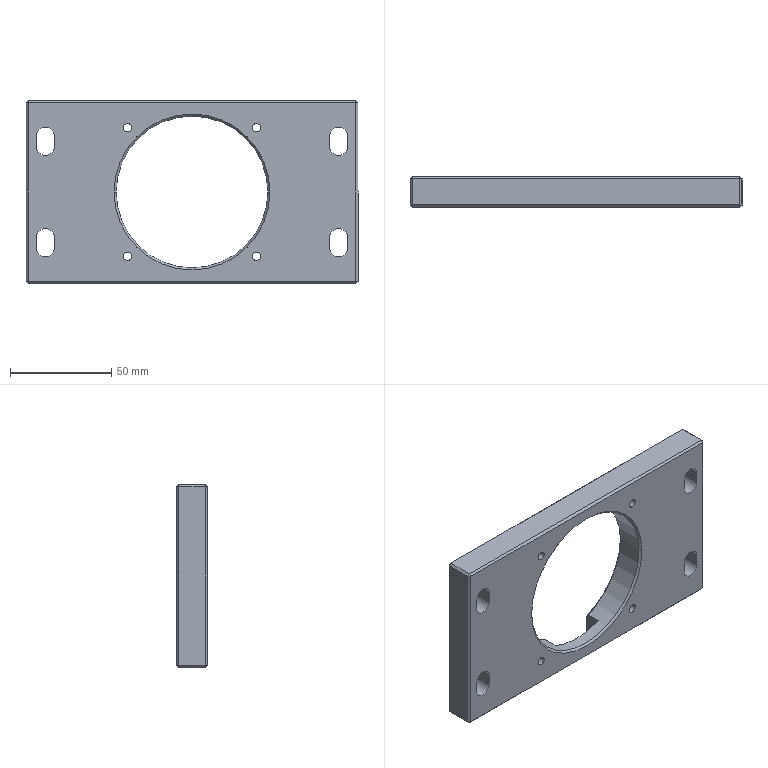Component | SolidWorks | ServoMotorFixingPlate-1 | 1 solid | 61 faces | box 164 x 15 x 90 mm | volume 144998 mm3 | plane 38 | cylinder 18 | cone 5 | commonest cylinder face diameters 4.2 x8 9 x8 75 x2 | material 1060 Alloy
build123d program:
from build123d import *

# Parameters (mm, degrees)
SKETCH1_W           = 164
SKETCH1_H           = 90
BOSS_EXTRUDE1_DEPTH = 15
CUT_EXTRUDE1_DEPTH  = 95.731
SKETCH7_R           = 37.5
CUT_EXTRUDE4_DEPTH  = 95.731
CHAMFER1_SIZE       = 1
M5_TAPPED_HOLE1_D   = 4.2
CIRPATTERN1_COUNT   = 4
SKETCH8_W           = 30
SKETCH8_H           = 14.214
CUT_EXTRUDE5_DEPTH  = 30


with BuildPart() as part:
    # Sketch1 → Boss-Extrude1 (new body)
    with BuildSketch(Plane.XY):
        Rectangle(SKETCH1_W, SKETCH1_H)
    extrude(amount=BOSS_EXTRUDE1_DEPTH)

    # Sketch2 → Cut-Extrude1 (cut, through all)
    with BuildSketch(Plane.XY.offset(15)):
        with BuildLine():
            Line((-68, 27.5), (-68, 22.5))
            ThreePointArc((-68, 22.5), (-72.5, 18), (-77, 22.5))
            Line((-77, 22.5), (-77, 27.5))
            ThreePointArc((-77, 27.5), (-72.5, 32), (-68, 27.5))
        make_face()
        with BuildLine():
            Line((-68, -22.5), (-68, -27.5))
            ThreePointArc((-68, -27.5), (-72.5, -32), (-77, -27.5))
            Line((-77, -27.5), (-77, -22.5))
            ThreePointArc((-77, -22.5), (-72.5, -18), (-68, -22.5))
        make_face()
        with BuildLine():
            Line((68, 22.5), (68, 27.5))
            ThreePointArc((68, 27.5), (72.5, 32), (77, 27.5))
            Line((77, 27.5), (77, 22.5))
            ThreePointArc((77, 22.5), (72.5, 18), (68, 22.5))
        make_face()
        with BuildLine():
            Line((68, -27.5), (68, -22.5))
            ThreePointArc((68, -22.5), (72.5, -18), (77, -22.5))
            Line((77, -22.5), (77, -27.5))
            ThreePointArc((77, -27.5), (72.5, -32), (68, -27.5))
        make_face()
    extrude(amount=-CUT_EXTRUDE1_DEPTH, mode=Mode.SUBTRACT)

    # Sketch7 → Cut-Extrude4 (cut, through all)
    with BuildSketch(Plane.XY.offset(15)):
        Circle(SKETCH7_R)
    extrude(amount=-CUT_EXTRUDE4_DEPTH, mode=Mode.SUBTRACT)

    # Chamfer1
    chamfer1_edges = [part.edges().sort_by_distance(p)[0] for p in [
        (82, 0, 15),
        (0, 45, 15),
        (-82, 0, 15),
        (0, 45, 0),
        (82, 0, 0),
        (0, -45, 0),
        (-82, 0, 0),
        (0, -45, 15),
        (-82, 45, 7.5),
        (82, 45, 7.5),
        (82, -45, 7.5),
        (-82, -45, 7.5),
        (-37.5, 0, 0),
        (-37.5, 0, 15),
    ]]
    chamfer(chamfer1_edges, length=CHAMFER1_SIZE)

    # M5 Tapped Hole1 (through all)
    with Locations(Plane.XY.offset(15)):
        with Locations((31.82, 31.82)):
            m5_tapped_hole1 = Hole(M5_TAPPED_HOLE1_D / 2)

    # CirPattern1: M5 Tapped Hole1 ×4 about axis
    cirpattern1_axis = Axis((0, 0, 0), (0, 0, 1))
    for i in range(1, CIRPATTERN1_COUNT):
        add(m5_tapped_hole1.rotate(cirpattern1_axis, i * 360 / CIRPATTERN1_COUNT), mode=Mode.SUBTRACT)

    # Sketch8 → Cut-Extrude5 (cut)
    with BuildSketch(Plane(origin=(0, -45, 0), x_dir=(1, 0, 0), z_dir=(0, 1, 0))):
        with Locations((0, -0.8928)):
            Rectangle(SKETCH8_W, SKETCH8_H)
    extrude(amount=CUT_EXTRUDE5_DEPTH, mode=Mode.SUBTRACT)


solid = part.part

# Placed as in the assembly
solid = solid.moved(Location((-47.166, 128.264, 99), (90, 0, 0)))